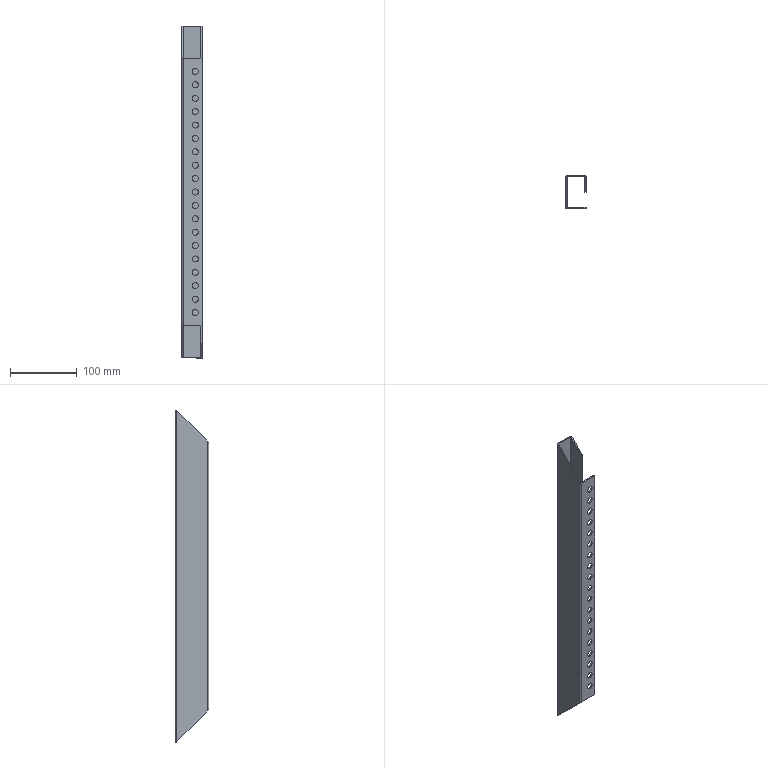Component | SolidWorks | KSHE-016.1.SLDPRT-1_KSHE-016.003-1 | 1 solid | 72 faces | volume 113204 mm3 | cylinder 44 | plane 28 | commonest cylinder face diameters 9 x38 4.2 x3 0.2 x3